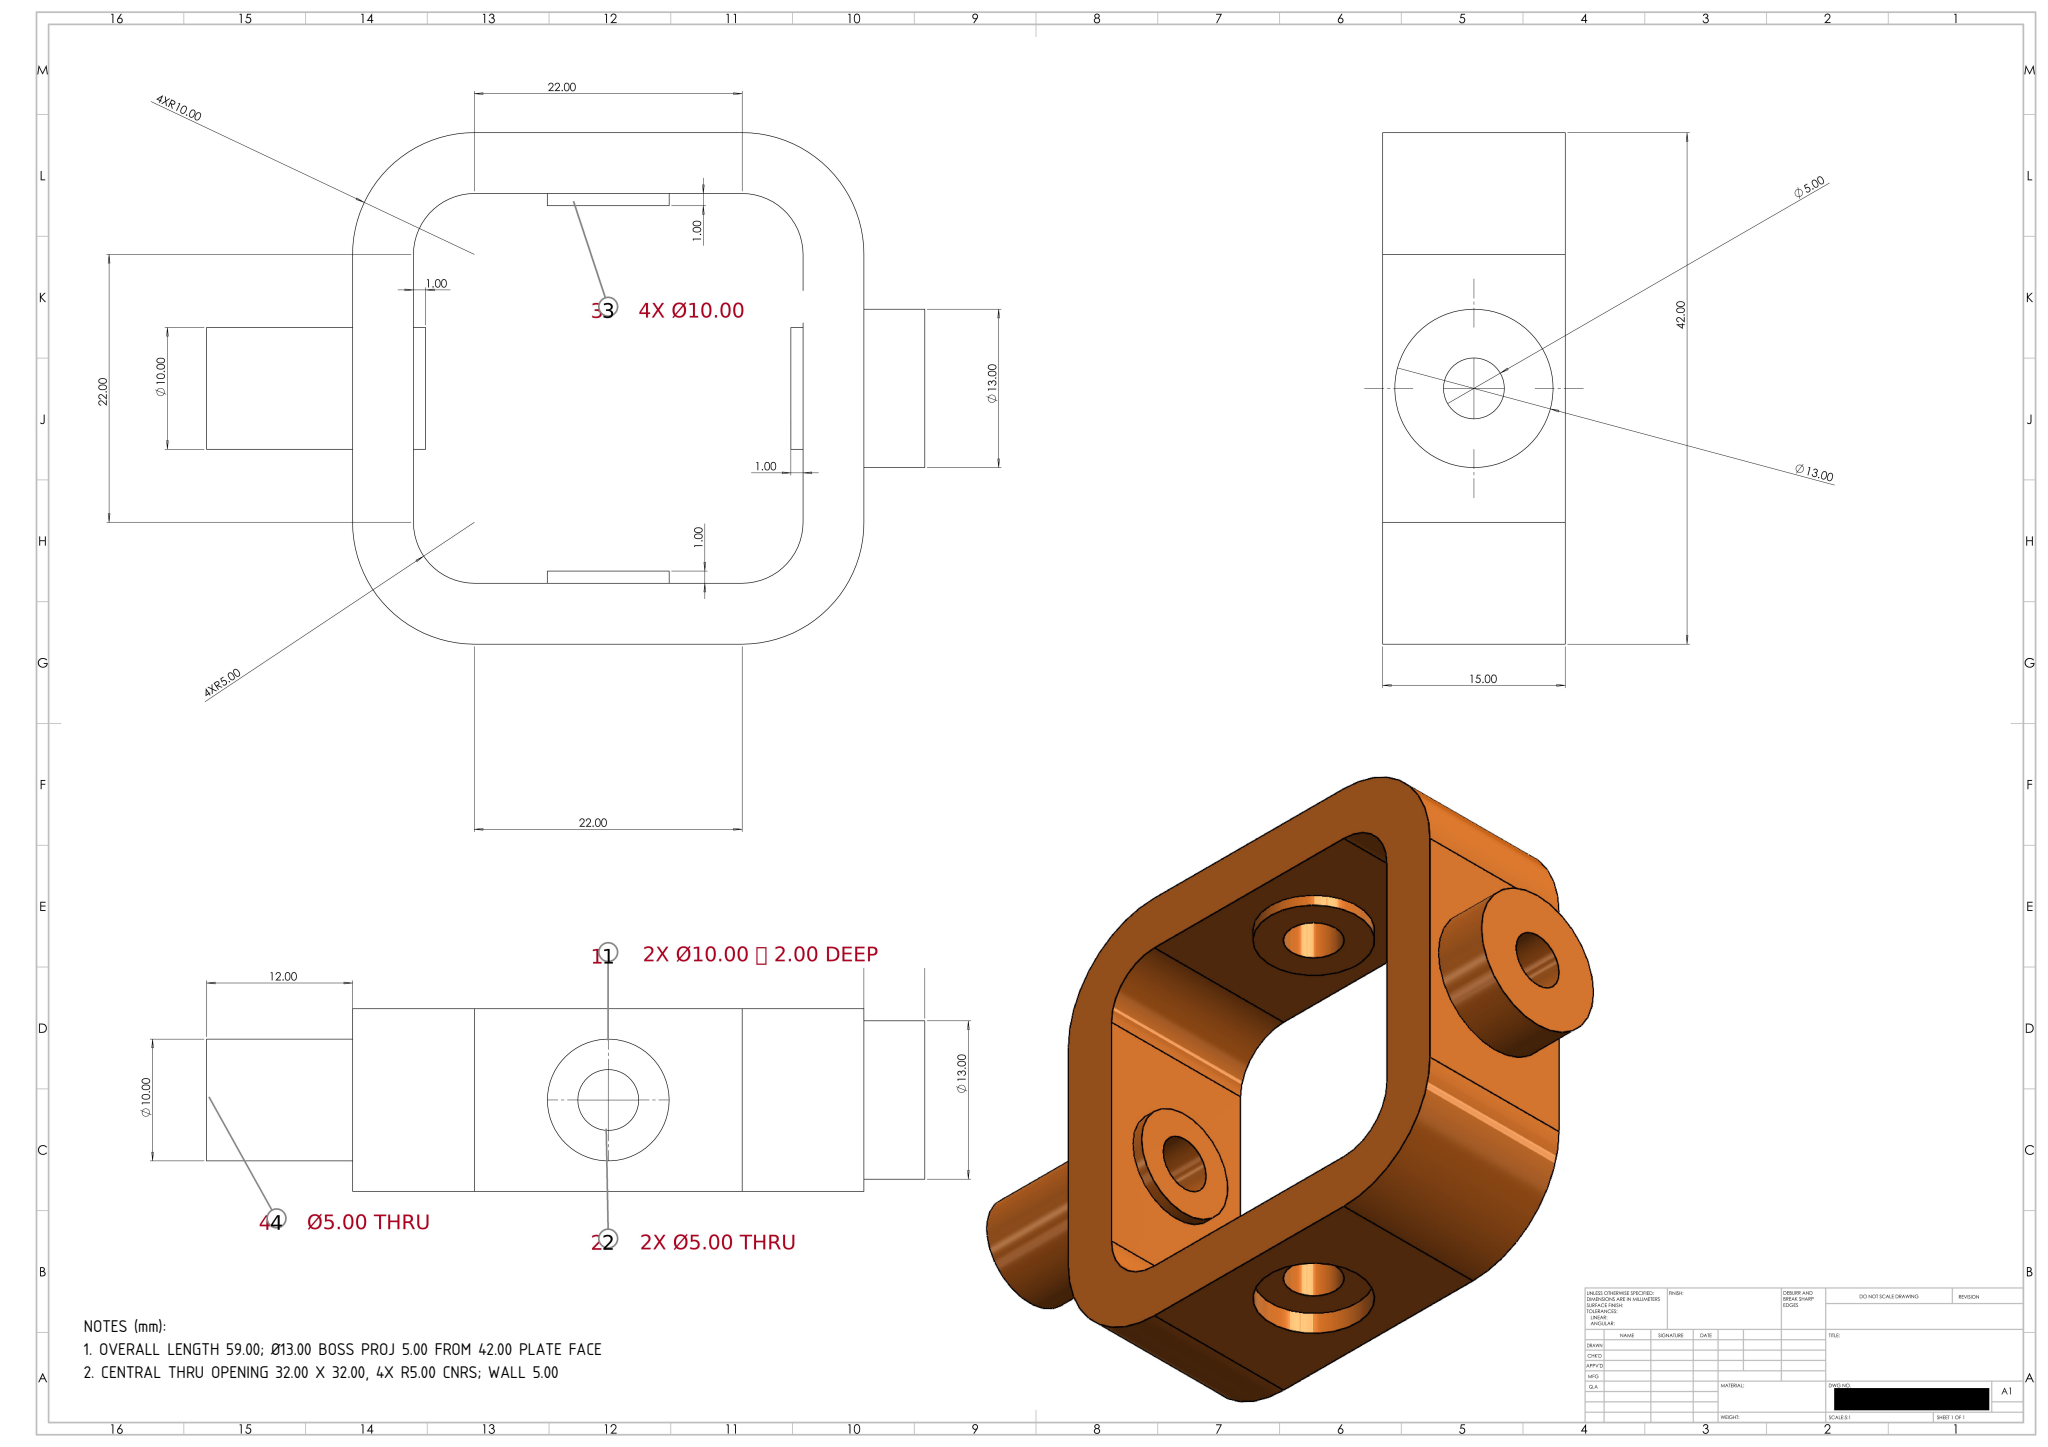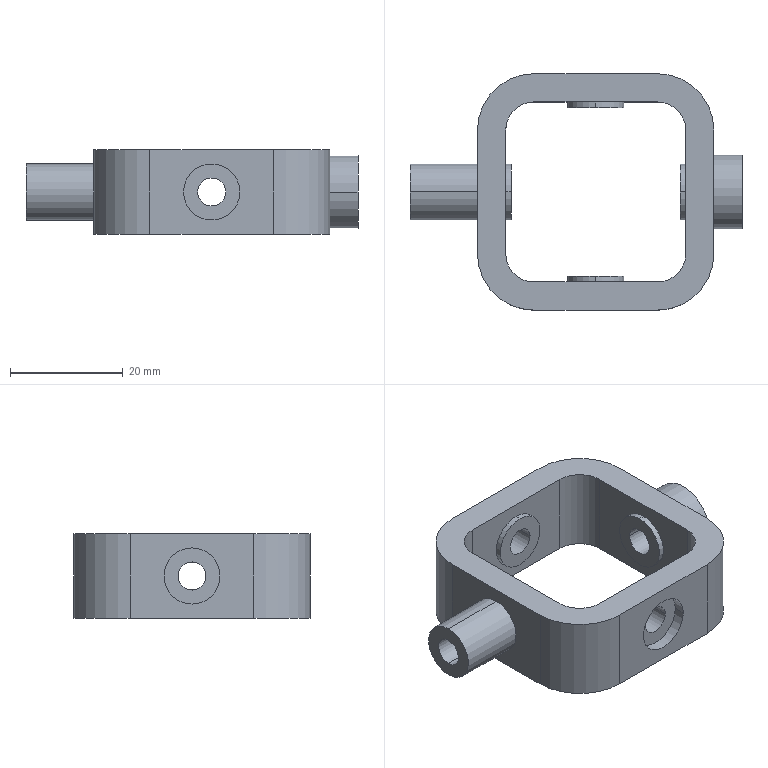Part | SolidWorks | mm | 1 solid | 50 faces | box 59 x 42 x 15 mm | volume 11014 mm3 | cylinder 32 | plane 18 | commonest cylinder face diameters 10 x18 5 x8 20 x4 13 x2
Drawing notes:
OVERALL LENGTH 59.00; Ø13.00 BOSS PROJ 5.00 FROM 42.00 PLATE FACE | from the solid: bbox_xyz X=59.0; plate faces at x=12.0 and x=54.0 (42.00 wide, set by R10 bosses at x=22/44); Ø13 x-axis cyl length 5.0 spanning x=54..59
CENTRAL THRU OPENING 32.00 X 32.00, 4X R5.00 CNRS; WALL 5.00 | from the solid: inner faces x=17.0/49.0 and y=5.0/37.0 give 32.00 x 32.00; outer faces x=12.0/54.0 and y=0/42.0 give 5.00 wall
build123d program:
from build123d import *

# Parameters (mm, degrees)
BOSS_EXTRUDE1_DEPTH = 15
SKETCH2_R           = 2.5
CUT_EXTRUDE1_DEPTH  = 50.318
SKETCH3_R           = 5
CUT_EXTRUDE2_DEPTH  = 2
CUT_EXTRUDE3_START  = -2
SKETCH4_R           = 5
CUT_EXTRUDE3_DEPTH  = 2
SKETCH5_R           = 5
SKETCH5_R_2         = 2.5
BOSS_EXTRUDE2_DEPTH = 1
BOSS_EXTRUDE3_START = 1
SKETCH6_R           = 5
SKETCH6_R_2         = 2.5
BOSS_EXTRUDE3_DEPTH = 1
SKETCH7_R           = 5
SKETCH7_R_2         = 2.5
BOSS_EXTRUDE4_DEPTH = 12
CUT_EXTRUDE4_START  = -12
SKETCH8_R           = 2.5
CUT_EXTRUDE4_DEPTH  = 12
BOSS_EXTRUDE5_START = 1
SKETCH9_R           = 5
SKETCH9_R_2         = 2.5
BOSS_EXTRUDE5_DEPTH = 1
BOSS_EXTRUDE6_START = 5
SKETCH10_R          = 6.5
SKETCH10_R_2        = 2.5
BOSS_EXTRUDE6_DEPTH = 5
SKETCH11_R          = 2.5
CUT_EXTRUDE5_DEPTH  = 8
SKETCH12_R          = 5
SKETCH12_R_2        = 2.5
BOSS_EXTRUDE7_DEPTH = 1


with BuildPart() as part:
    # Sketch1 → Boss-Extrude1 (new body)
    with BuildSketch(Plane.XY):
        with BuildLine():
            Line((-11.055, -20.891), (-0.05464, -20.891))
            Line((-0.05464, -20.891), (10.945, -20.891))
            ThreePointArc((10.945, -20.891), (18.016, -17.962), (20.945, -10.891))
            Line((20.945, -10.891), (20.945, 11.109))
            ThreePointArc((20.945, 11.109), (18.016, 18.18), (10.945, 21.109))
            Line((10.945, 21.109), (-11.055, 21.109))
            ThreePointArc((-11.055, 21.109), (-18.126, 18.18), (-21.055, 11.109))
            Line((-21.055, 11.109), (-21.055, -10.891))
            ThreePointArc((-21.055, -10.891), (-18.126, -17.962), (-11.055, -20.891))
        make_face()
        with BuildLine():
            Line((15.945, -10.891), (15.945, 11.109))
            ThreePointArc((15.945, 11.109), (14.481, 14.645), (10.945, 16.109))
            Line((10.945, 16.109), (-11.055, 16.109))
            ThreePointArc((-11.055, 16.109), (-14.59, 14.645), (-16.055, 11.109))
            Line((-16.055, 11.109), (-16.055, -10.891))
            ThreePointArc((-16.055, -10.891), (-14.59, -14.426), (-11.055, -15.891))
            Line((-11.055, -15.891), (10.945, -15.891))
            ThreePointArc((10.945, -15.891), (14.481, -14.426), (15.945, -10.891))
        make_face(mode=Mode.SUBTRACT)
    extrude(amount=BOSS_EXTRUDE1_DEPTH)

    # Sketch2 → Cut-Extrude1 (cut, through all)
    with BuildSketch(Plane.XZ.offset(20.891)):
        with Locations((-0.05464, 7.5)):
            Circle(SKETCH2_R)
    extrude(amount=-CUT_EXTRUDE1_DEPTH, mode=Mode.SUBTRACT)

    # Sketch3 → Cut-Extrude2 (cut)
    with BuildSketch(Plane.XZ.offset(20.891)):
        with Locations((-0.05464, 7.5)):
            Circle(SKETCH3_R)
    extrude(amount=-CUT_EXTRUDE2_DEPTH, mode=Mode.SUBTRACT)

    # Sketch4 → Cut-Extrude3 (cut)
    with BuildSketch(Plane(origin=(0, 21.109, 0), x_dir=(1, 0, 0), z_dir=(0, 1, 0)).offset(CUT_EXTRUDE3_START)):
        with Locations((-0.05464, -7.5)):
            Circle(SKETCH4_R)
    extrude(amount=CUT_EXTRUDE3_DEPTH, mode=Mode.SUBTRACT)

    # Sketch5 → Boss-Extrude2 (add)
    with BuildSketch(Plane(origin=(0, -15.891, 0), x_dir=(1, 0, 0), z_dir=(0, 1, 0))):
        with Locations((-0.05464, -7.5)):
            Circle(SKETCH5_R)
        with Locations((-0.05464, -7.5)):
            Circle(SKETCH5_R_2, mode=Mode.SUBTRACT)
    extrude(amount=BOSS_EXTRUDE2_DEPTH)

    # Sketch6 → Boss-Extrude3 (add)
    with BuildSketch(Plane.XZ.offset(-16.109).offset(BOSS_EXTRUDE3_START)):
        with Locations((-0.05464, 7.5)):
            Circle(SKETCH6_R)
        with Locations((-0.05464, 7.5)):
            Circle(SKETCH6_R_2, mode=Mode.SUBTRACT)
    extrude(amount=-BOSS_EXTRUDE3_DEPTH)

    # Sketch7 → Boss-Extrude4 (add)
    with BuildSketch(Plane.ZY.offset(21.055)):
        with Locations(Location((7.5, 0.1093, 0), (0, 0, 180))):
            Circle(SKETCH7_R)
        with Locations((7.5, 0.1093)):
            Circle(SKETCH7_R_2, mode=Mode.SUBTRACT)
    extrude(amount=BOSS_EXTRUDE4_DEPTH)

    # Sketch8 → Cut-Extrude4 (cut)
    with BuildSketch(Plane.ZY.offset(21.055).offset(CUT_EXTRUDE4_START)):
        with Locations(Location((7.5, 0.1093, 0), (0, 0, 180))):
            Circle(SKETCH8_R)
    extrude(amount=CUT_EXTRUDE4_DEPTH, mode=Mode.SUBTRACT)

    # Sketch9 → Boss-Extrude5 (add)
    with BuildSketch(Plane(origin=(-16.055, 0, 0), x_dir=(0, 0, -1), z_dir=(1, 0, 0)).offset(BOSS_EXTRUDE5_START)):
        with Locations((-7.5, 0.1093)):
            Circle(SKETCH9_R)
        with Locations((-7.5, 0.1093)):
            Circle(SKETCH9_R_2, mode=Mode.SUBTRACT)
    extrude(amount=-BOSS_EXTRUDE5_DEPTH)

    # Sketch10 → Boss-Extrude6 (add)
    with BuildSketch(Plane(origin=(20.945, 0, 0), x_dir=(0, 0, -1), z_dir=(1, 0, 0)).offset(BOSS_EXTRUDE6_START)):
        with Locations(Location((-7.5, 0.1093, 0), (0, 0, 270))):
            Circle(SKETCH10_R)
        with Locations((-7.5, 0.1093)):
            Circle(SKETCH10_R_2, mode=Mode.SUBTRACT)
    extrude(amount=-BOSS_EXTRUDE6_DEPTH)

    # Sketch11 → Cut-Extrude5 (cut)
    with BuildSketch(Plane(origin=(20.945, 0, 0), x_dir=(0, 0, -1), z_dir=(1, 0, 0))):
        with Locations((-7.5, 0.1093)):
            Circle(SKETCH11_R)
    extrude(amount=-CUT_EXTRUDE5_DEPTH, mode=Mode.SUBTRACT)

    # Sketch12 → Boss-Extrude7 (add)
    with BuildSketch(Plane.ZY.offset(-15.945)):
        with Locations(Location((7.5, 0.1093, 0), (0, 0, 180))):
            Circle(SKETCH12_R)
        with Locations(Location((7.5, 0.1093, 0), (0, 0, 180))):
            Circle(SKETCH12_R_2, mode=Mode.SUBTRACT)
    extrude(amount=BOSS_EXTRUDE7_DEPTH)


solid = part.part